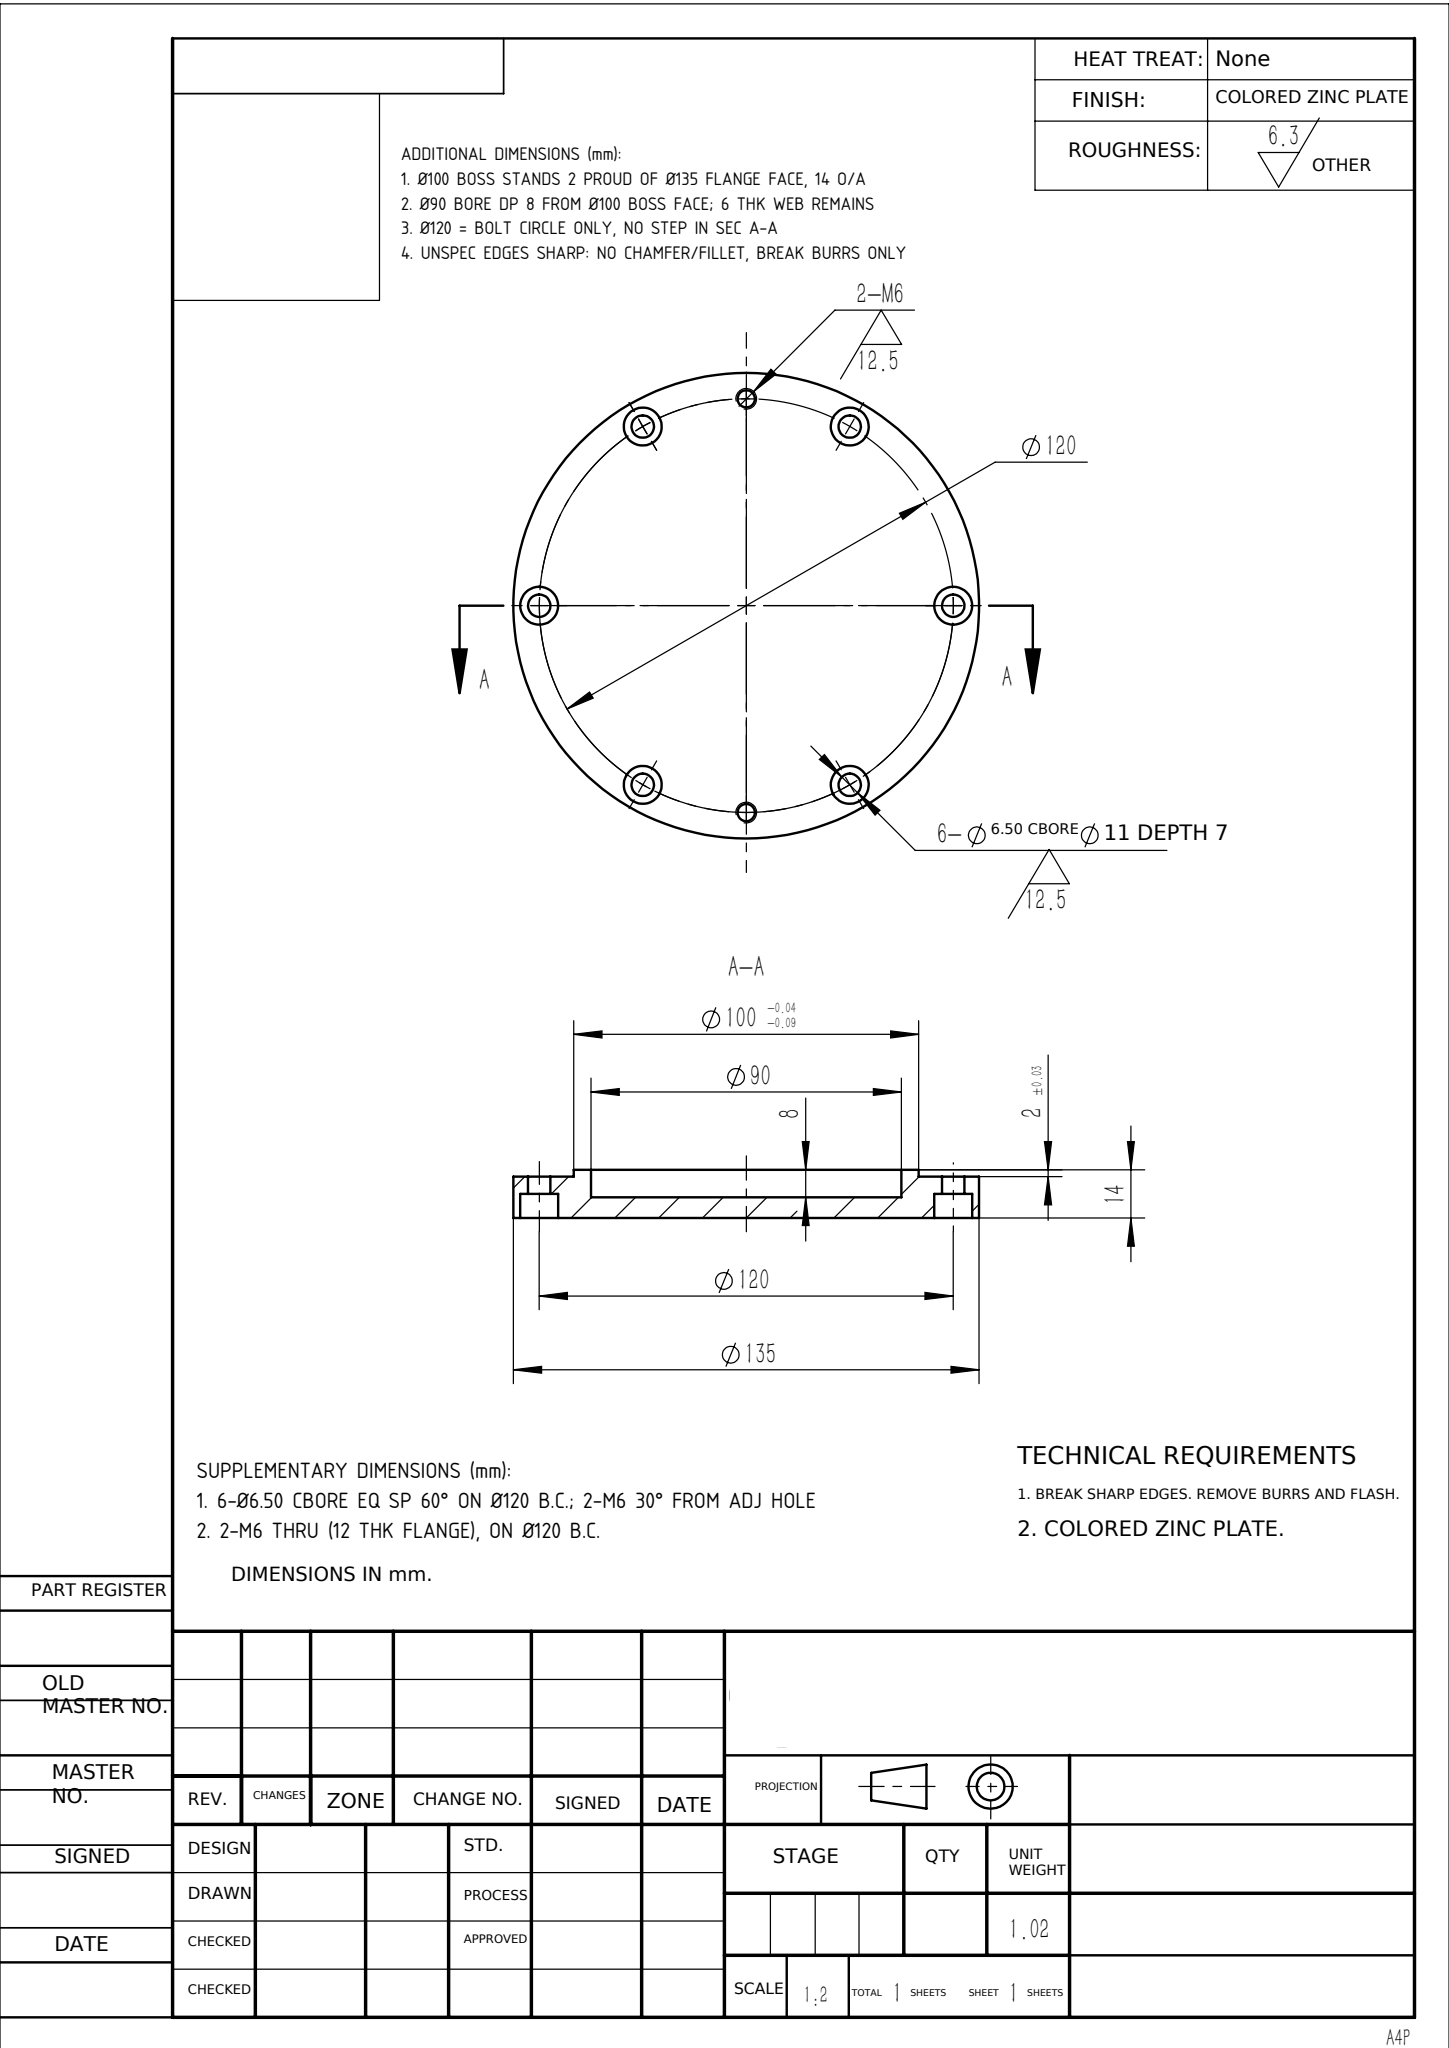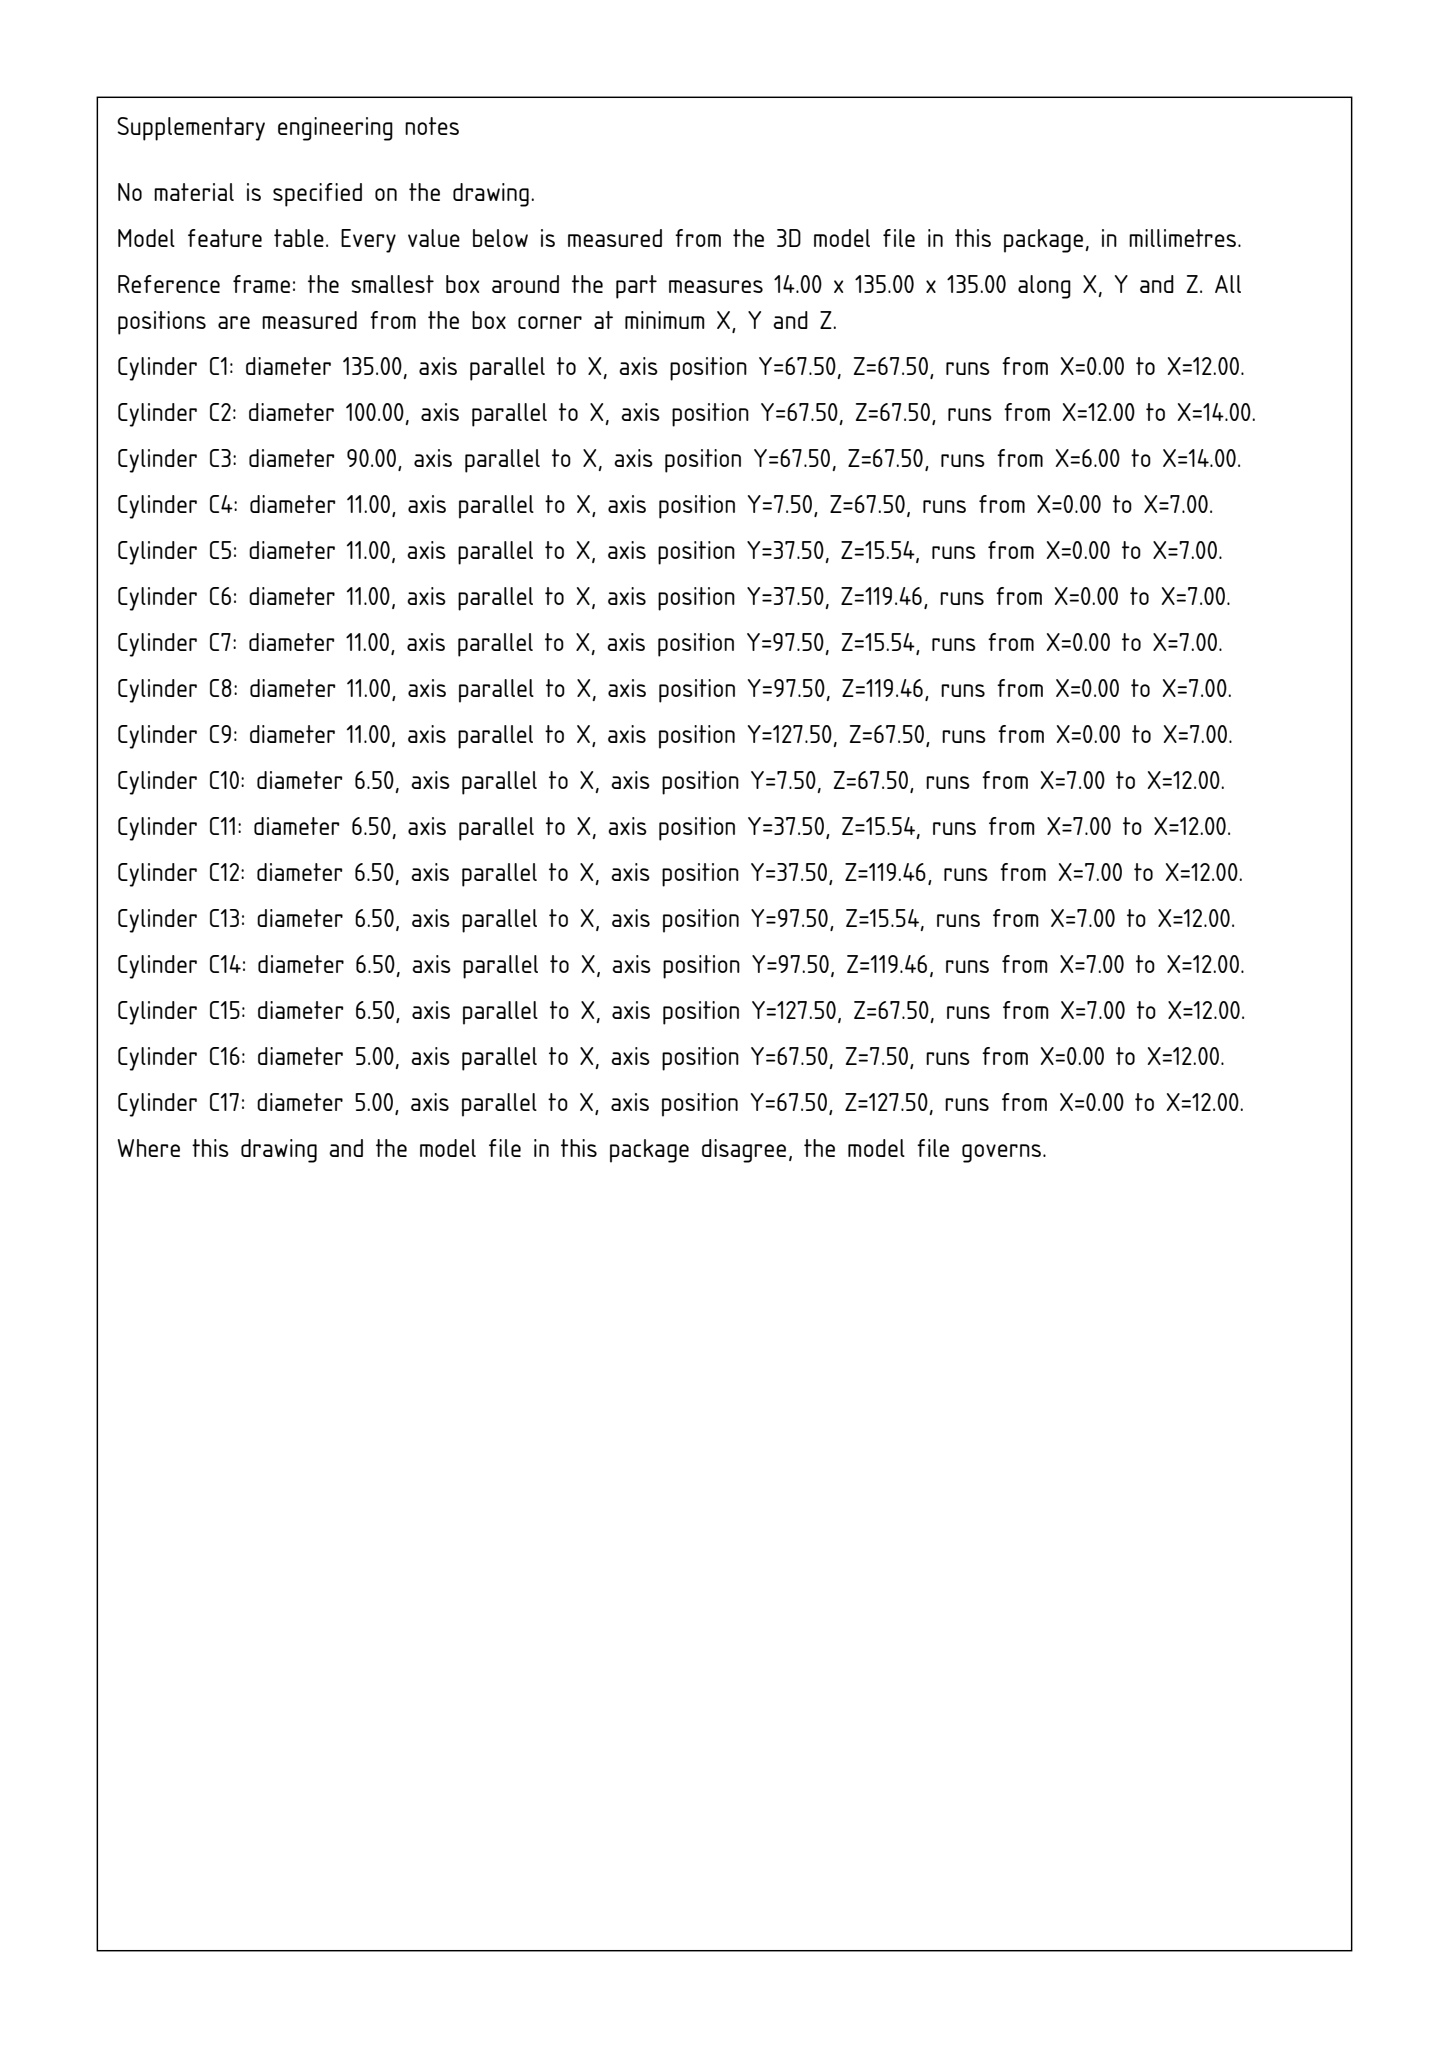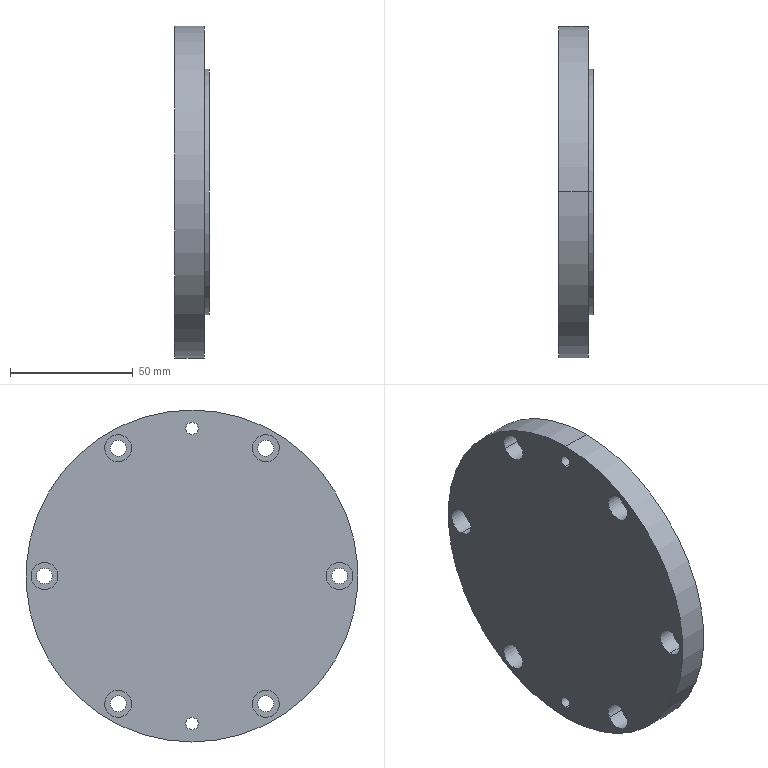Part | SolidWorks | mm | 1 solid | 44 faces | box 14 x 135 x 135 mm | volume 131123 mm3 | cylinder 34 | plane 10 | commonest cylinder face diameters 11 x12 6.5 x12 5 x4 135 x2 100 x2 90 x2
build123d program:
from build123d import *

# Parameters (mm, degrees)
SKETCH2_R          = 3.25
CUT_EXTRUDE1_DEPTH = 97.211
SKETCH3_R          = 5.5
CUT_EXTRUDE2_DEPTH = 7
CIRPATTERN1_COUNT  = 6
M6_TAPPED_HOLE1_D  = 5
CIRPATTERN2_COUNT  = 2


with BuildPart() as part:
    # Sketch1 → Revolve1 (revolve)
    with BuildSketch(Plane.XY, mode=Mode.PRIVATE) as revolve1_sk:
        Polygon((0, 0), (6, 0), (6, 45), (14, 45), (14, 50), (12, 50), (12, 67.5), (0, 67.5), align=None)
    revolve(revolve1_sk.sketch.rotate(Axis((0, 0, 0), (1, 0, 0)), 90), axis=Axis((0, 0, 0), (1, 0, 0)))

    # Sketch2 → Cut-Extrude1 (cut, through all)
    with BuildSketch(Plane(origin=(12, 0, 0), x_dir=(0, 0, -1), z_dir=(1, 0, 0))):
        with Locations((0, 60)):
            Circle(SKETCH2_R)
    cut_extrude1 = extrude(amount=-CUT_EXTRUDE1_DEPTH, mode=Mode.SUBTRACT)

    # Sketch3 → Cut-Extrude2 (cut)
    with BuildSketch(Plane.ZY):
        with Locations((0, 60)):
            Circle(SKETCH3_R)
    cut_extrude2 = extrude(amount=-CUT_EXTRUDE2_DEPTH, mode=Mode.SUBTRACT)

    # CirPattern1: Cut-Extrude1, Cut-Extrude2 ×6 about axis
    cirpattern1_axis = Axis((0, 0, 0), (1, 0, 0))
    add([cut_extrude1.rotate(cirpattern1_axis, i * 360 / CIRPATTERN1_COUNT) for i in range(1, CIRPATTERN1_COUNT)], mode=Mode.SUBTRACT)
    add([cut_extrude2.rotate(cirpattern1_axis, i * 360 / CIRPATTERN1_COUNT) for i in range(1, CIRPATTERN1_COUNT)], mode=Mode.SUBTRACT)

    # M6 Tapped Hole1 (through all)
    with Locations(Plane.ZY):
        with Locations((-60, 0)):
            m6_tapped_hole1 = Hole(M6_TAPPED_HOLE1_D / 2)

    # CirPattern2: M6 Tapped Hole1 ×2 about axis
    cirpattern2_axis = Axis((0, 0, 0), (1, 0, 0))
    for i in range(1, CIRPATTERN2_COUNT):
        add(m6_tapped_hole1.rotate(cirpattern2_axis, i * 360 / CIRPATTERN2_COUNT), mode=Mode.SUBTRACT)


solid = part.part